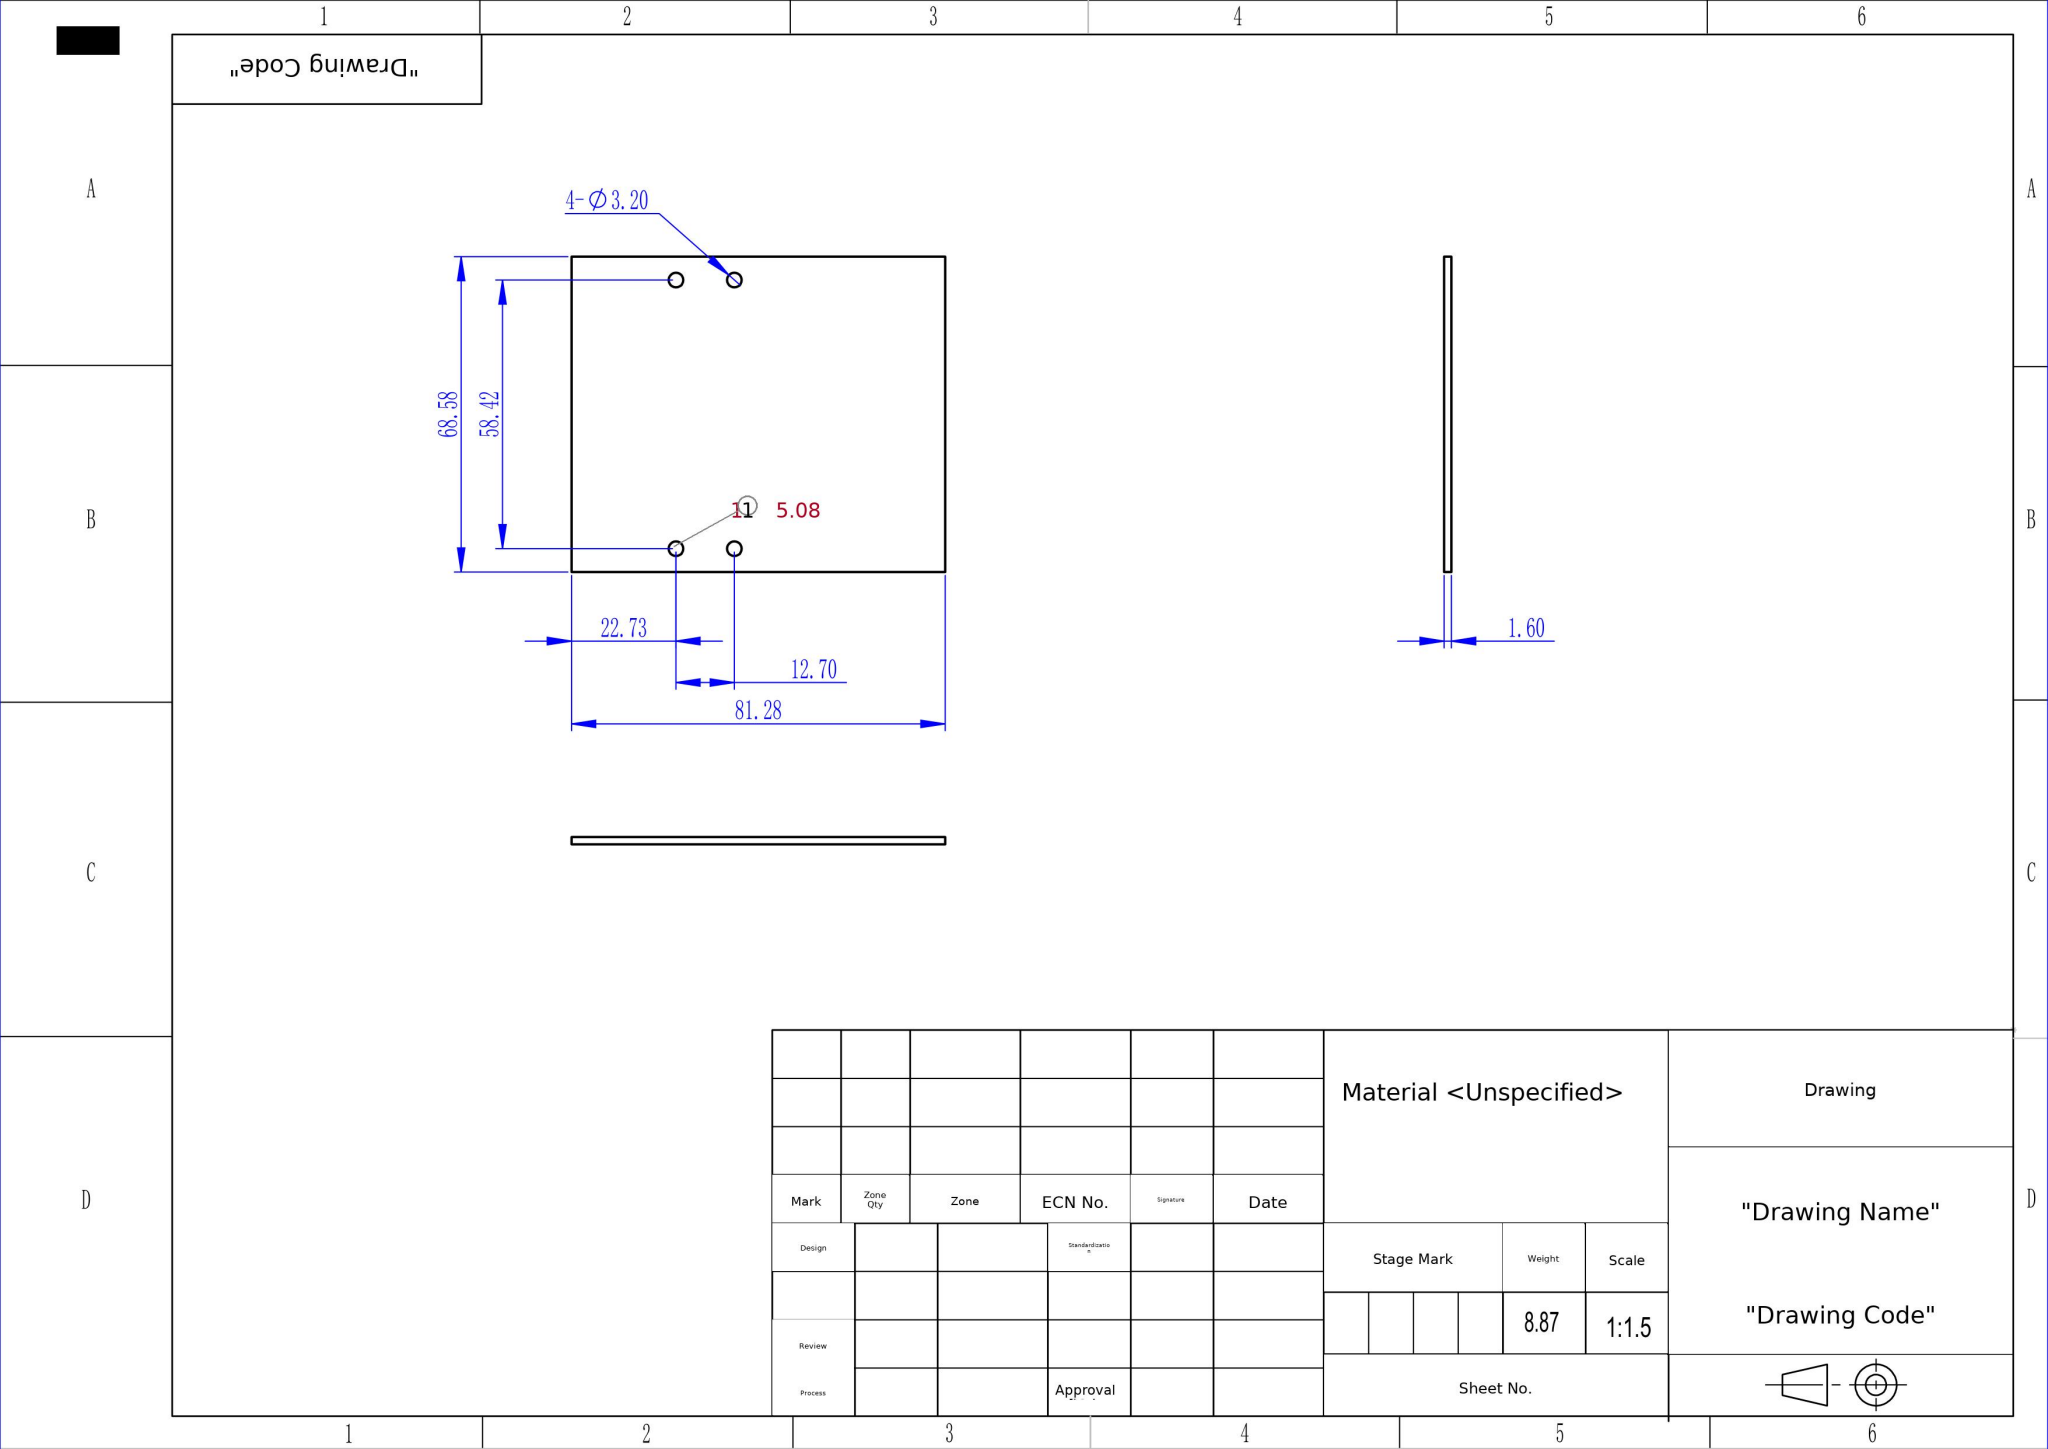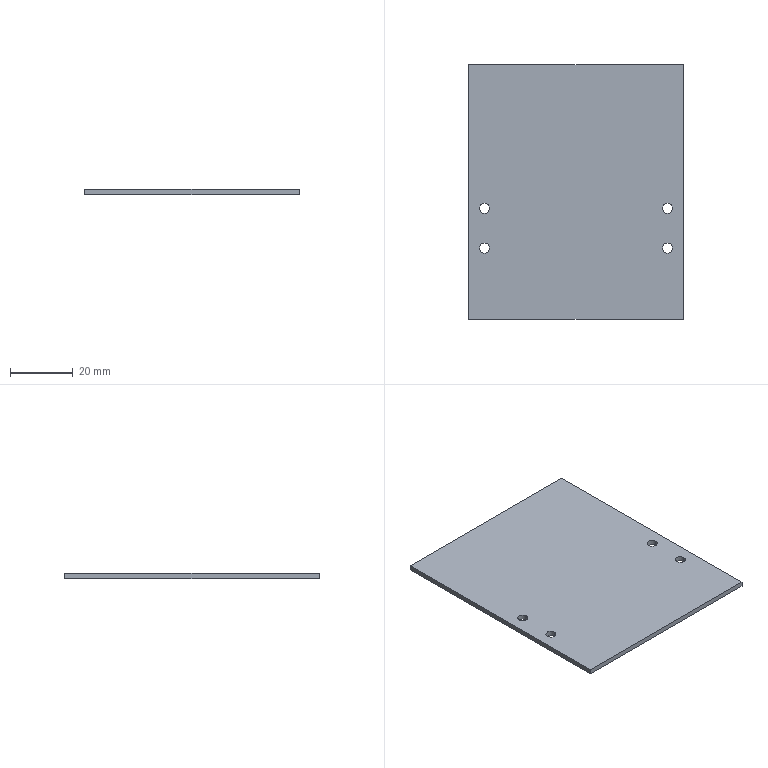Part | SolidWorks | mm | material Unspecified | 1 solid | 14 faces | box 68.58 x 81.28 x 1.6 mm | volume 8867 mm3 | cylinder 8 | plane 6 | commonest cylinder face diameters 3.2 x8
build123d program:
from build123d import *

# Parameters (mm, degrees)
SKETCH1_W           = 68.58
SKETCH1_H           = 81.28
SKETCH1_R           = 1.6
BOSS_EXTRUDE1_DEPTH = 1.6


with BuildPart() as part:
    # Sketch1 → Boss-Extrude1 (new body)
    with BuildSketch(Plane.XY):
        with Locations((0, 11.56)):
            Rectangle(SKETCH1_W, SKETCH1_H)
        with Locations((-29.21, 6.35)):
            Circle(SKETCH1_R, mode=Mode.SUBTRACT)
        with Locations((29.21, 6.35)):
            Circle(SKETCH1_R, mode=Mode.SUBTRACT)
        with Locations((29.21, -6.35)):
            Circle(SKETCH1_R, mode=Mode.SUBTRACT)
        with Locations((-29.21, -6.35)):
            Circle(SKETCH1_R, mode=Mode.SUBTRACT)
    extrude(amount=BOSS_EXTRUDE1_DEPTH)


solid = part.part
STEP:
#1=CARTESIAN_POINT('',(-30.81,-6.35,1.6));
#2=VERTEX_POINT('',#1);
#3=CARTESIAN_POINT('',(-27.61,-6.35,1.6));
#4=VERTEX_POINT('',#3);
#5=CARTESIAN_POINT('',(-29.21,-6.35,1.6));
#6=DIRECTION('',(0.,0.,1.));
#7=DIRECTION('',(1.,0.,0.));
#8=AXIS2_PLACEMENT_3D('',#5,#6,#7);
#9=CIRCLE('',#8,1.6);
#10=EDGE_CURVE('',#2,#4,#9,.T.);
#11=ORIENTED_EDGE('',*,*,#10,.T.);
#12=CARTESIAN_POINT('',(-27.61,-6.35,0.));
#13=VERTEX_POINT('',#12);
#14=CARTESIAN_POINT('',(-27.61,-6.35,1.6));
#15=DIRECTION('',(0.,0.,-1.));
#16=VECTOR('',#15,1000.);
#17=LINE('',#14,#16);
#18=EDGE_CURVE('',#4,#13,#17,.T.);
#19=ORIENTED_EDGE('',*,*,#18,.T.);
#20=CARTESIAN_POINT('',(-30.81,-6.35,0.));
#21=VERTEX_POINT('',#20);
#22=CARTESIAN_POINT('',(-29.21,-6.35,0.));
#23=DIRECTION('',(0.,0.,1.));
#24=DIRECTION('',(1.,0.,0.));
#25=AXIS2_PLACEMENT_3D('',#22,#23,#24);
#26=CIRCLE('',#25,1.6);
#27=EDGE_CURVE('',#21,#13,#26,.T.);
#28=ORIENTED_EDGE('',*,*,#27,.F.);
#29=CARTESIAN_POINT('',(-30.81,-6.35,1.6));
#30=DIRECTION('',(0.,0.,-1.));
#31=VECTOR('',#30,1000.);
#32=LINE('',#29,#31);
#33=EDGE_CURVE('',#2,#21,#32,.T.);
#34=ORIENTED_EDGE('',*,*,#33,.F.);
#35=EDGE_LOOP('',(#11,#19,#28,#34));
#36=FACE_OUTER_BOUND('',#35,.T.);
#37=CARTESIAN_POINT('',(-29.21,-6.35,1.6));
#38=DIRECTION('',(0.,0.,-1.));
#39=DIRECTION('',(-1.,0.,0.));
#40=AXIS2_PLACEMENT_3D('',#37,#38,#39);
#41=CYLINDRICAL_SURFACE('',#40,1.6);
#42=ADVANCED_FACE('',(#36),#41,.F.);
#43=CARTESIAN_POINT('',(27.61,-6.35,1.6));
#44=VERTEX_POINT('',#43);
#45=CARTESIAN_POINT('',(30.81,-6.35,1.6));
#46=VERTEX_POINT('',#45);
#47=CARTESIAN_POINT('',(29.21,-6.35,1.6));
#48=DIRECTION('',(0.,0.,1.));
#49=DIRECTION('',(1.,0.,0.));
#50=AXIS2_PLACEMENT_3D('',#47,#48,#49);
#51=CIRCLE('',#50,1.6);
#52=EDGE_CURVE('',#44,#46,#51,.T.);
#53=ORIENTED_EDGE('',*,*,#52,.T.);
#54=CARTESIAN_POINT('',(30.81,-6.35,0.));
#55=VERTEX_POINT('',#54);
#56=CARTESIAN_POINT('',(30.81,-6.35,1.6));
#57=DIRECTION('',(0.,0.,-1.));
#58=VECTOR('',#57,1000.);
#59=LINE('',#56,#58);
#60=EDGE_CURVE('',#46,#55,#59,.T.);
#61=ORIENTED_EDGE('',*,*,#60,.T.);
#62=CARTESIAN_POINT('',(27.61,-6.35,0.));
#63=VERTEX_POINT('',#62);
#64=CARTESIAN_POINT('',(29.21,-6.35,0.));
#65=DIRECTION('',(0.,0.,1.));
#66=DIRECTION('',(1.,0.,0.));
#67=AXIS2_PLACEMENT_3D('',#64,#65,#66);
#68=CIRCLE('',#67,1.6);
#69=EDGE_CURVE('',#63,#55,#68,.T.);
#70=ORIENTED_EDGE('',*,*,#69,.F.);
#71=CARTESIAN_POINT('',(27.61,-6.35,1.6));
#72=DIRECTION('',(0.,0.,-1.));
#73=VECTOR('',#72,1000.);
#74=LINE('',#71,#73);
#75=EDGE_CURVE('',#44,#63,#74,.T.);
#76=ORIENTED_EDGE('',*,*,#75,.F.);
#77=EDGE_LOOP('',(#53,#61,#70,#76));
#78=FACE_OUTER_BOUND('',#77,.T.);
#79=CARTESIAN_POINT('',(29.21,-6.35,1.6));
#80=DIRECTION('',(0.,0.,-1.));
#81=DIRECTION('',(-1.,0.,0.));
#82=AXIS2_PLACEMENT_3D('',#79,#80,#81);
#83=CYLINDRICAL_SURFACE('',#82,1.6);
#84=ADVANCED_FACE('',(#78),#83,.F.);
#85=CARTESIAN_POINT('',(27.61,6.35,1.6));
#86=VERTEX_POINT('',#85);
#87=CARTESIAN_POINT('',(30.81,6.35,1.6));
#88=VERTEX_POINT('',#87);
#89=CARTESIAN_POINT('',(29.21,6.35,1.6));
#90=DIRECTION('',(0.,0.,1.));
#91=DIRECTION('',(1.,0.,0.));
#92=AXIS2_PLACEMENT_3D('',#89,#90,#91);
#93=CIRCLE('',#92,1.6);
#94=EDGE_CURVE('',#86,#88,#93,.T.);
#95=ORIENTED_EDGE('',*,*,#94,.T.);
#96=CARTESIAN_POINT('',(30.81,6.35,0.));
#97=VERTEX_POINT('',#96);
#98=CARTESIAN_POINT('',(30.81,6.35,1.6));
#99=DIRECTION('',(0.,0.,-1.));
#100=VECTOR('',#99,1000.);
#101=LINE('',#98,#100);
#102=EDGE_CURVE('',#88,#97,#101,.T.);
#103=ORIENTED_EDGE('',*,*,#102,.T.);
#104=CARTESIAN_POINT('',(27.61,6.35,0.));
#105=VERTEX_POINT('',#104);
#106=CARTESIAN_POINT('',(29.21,6.35,0.));
#107=DIRECTION('',(0.,0.,1.));
#108=DIRECTION('',(1.,0.,0.));
#109=AXIS2_PLACEMENT_3D('',#106,#107,#108);
#110=CIRCLE('',#109,1.6);
#111=EDGE_CURVE('',#105,#97,#110,.T.);
#112=ORIENTED_EDGE('',*,*,#111,.F.);
#113=CARTESIAN_POINT('',(27.61,6.35,1.6));
#114=DIRECTION('',(0.,0.,-1.));
#115=VECTOR('',#114,1000.);
#116=LINE('',#113,#115);
#117=EDGE_CURVE('',#86,#105,#116,.T.);
#118=ORIENTED_EDGE('',*,*,#117,.F.);
#119=EDGE_LOOP('',(#95,#103,#112,#118));
#120=FACE_OUTER_BOUND('',#119,.T.);
#121=CARTESIAN_POINT('',(29.21,6.35,1.6));
#122=DIRECTION('',(0.,0.,-1.));
#123=DIRECTION('',(-1.,0.,0.));
#124=AXIS2_PLACEMENT_3D('',#121,#122,#123);
#125=CYLINDRICAL_SURFACE('',#124,1.6);
#126=ADVANCED_FACE('',(#120),#125,.F.);
#127=CARTESIAN_POINT('',(-30.81,6.35,1.6));
#128=VERTEX_POINT('',#127);
#129=CARTESIAN_POINT('',(-27.61,6.35,1.6));
#130=VERTEX_POINT('',#129);
#131=CARTESIAN_POINT('',(-29.21,6.35,1.6));
#132=DIRECTION('',(0.,0.,1.));
#133=DIRECTION('',(1.,0.,0.));
#134=AXIS2_PLACEMENT_3D('',#131,#132,#133);
#135=CIRCLE('',#134,1.6);
#136=EDGE_CURVE('',#128,#130,#135,.T.);
#137=ORIENTED_EDGE('',*,*,#136,.T.);
#138=CARTESIAN_POINT('',(-27.61,6.35,0.));
#139=VERTEX_POINT('',#138);
#140=CARTESIAN_POINT('',(-27.61,6.35,1.6));
#141=DIRECTION('',(0.,0.,-1.));
#142=VECTOR('',#141,1000.);
#143=LINE('',#140,#142);
#144=EDGE_CURVE('',#130,#139,#143,.T.);
#145=ORIENTED_EDGE('',*,*,#144,.T.);
#146=CARTESIAN_POINT('',(-30.81,6.35,0.));
#147=VERTEX_POINT('',#146);
#148=CARTESIAN_POINT('',(-29.21,6.35,0.));
#149=DIRECTION('',(0.,0.,1.));
#150=DIRECTION('',(1.,0.,0.));
#151=AXIS2_PLACEMENT_3D('',#148,#149,#150);
#152=CIRCLE('',#151,1.6);
#153=EDGE_CURVE('',#147,#139,#152,.T.);
#154=ORIENTED_EDGE('',*,*,#153,.F.);
#155=CARTESIAN_POINT('',(-30.81,6.35,1.6));
#156=DIRECTION('',(0.,0.,-1.));
#157=VECTOR('',#156,1000.);
#158=LINE('',#155,#157);
#159=EDGE_CURVE('',#128,#147,#158,.T.);
#160=ORIENTED_EDGE('',*,*,#159,.F.);
#161=EDGE_LOOP('',(#137,#145,#154,#160));
#162=FACE_OUTER_BOUND('',#161,.T.);
#163=CARTESIAN_POINT('',(-29.21,6.35,1.6));
#164=DIRECTION('',(0.,0.,-1.));
#165=DIRECTION('',(-1.,0.,0.));
#166=AXIS2_PLACEMENT_3D('',#163,#164,#165);
#167=CYLINDRICAL_SURFACE('',#166,1.6);
#168=ADVANCED_FACE('',(#162),#167,.F.);
#169=CARTESIAN_POINT('',(34.29,-29.08,1.6));
#170=VERTEX_POINT('',#169);
#171=CARTESIAN_POINT('',(34.29,52.2,1.6));
#172=VERTEX_POINT('',#171);
#173=CARTESIAN_POINT('',(34.29,-29.08,1.6));
#174=DIRECTION('',(0.,1.,0.));
#175=VECTOR('',#174,1000.);
#176=LINE('',#173,#175);
#177=EDGE_CURVE('',#170,#172,#176,.T.);
#178=ORIENTED_EDGE('',*,*,#177,.T.);
#179=CARTESIAN_POINT('',(-34.29,52.2,1.6));
#180=VERTEX_POINT('',#179);
#181=CARTESIAN_POINT('',(-34.29,52.2,1.6));
#182=DIRECTION('',(-1.,0.,0.));
#183=VECTOR('',#182,1000.);
#184=LINE('',#181,#183);
#185=EDGE_CURVE('',#172,#180,#184,.T.);
#186=ORIENTED_EDGE('',*,*,#185,.T.);
#187=CARTESIAN_POINT('',(-34.29,-29.08,1.6));
#188=VERTEX_POINT('',#187);
#189=CARTESIAN_POINT('',(-34.29,-29.08,1.6));
#190=DIRECTION('',(0.,-1.,0.));
#191=VECTOR('',#190,1000.);
#192=LINE('',#189,#191);
#193=EDGE_CURVE('',#180,#188,#192,.T.);
#194=ORIENTED_EDGE('',*,*,#193,.T.);
#195=CARTESIAN_POINT('',(-34.29,-29.08,1.6));
#196=DIRECTION('',(1.,0.,0.));
#197=VECTOR('',#196,1000.);
#198=LINE('',#195,#197);
#199=EDGE_CURVE('',#188,#170,#198,.T.);
#200=ORIENTED_EDGE('',*,*,#199,.T.);
#201=EDGE_LOOP('',(#178,#186,#194,#200));
#202=FACE_OUTER_BOUND('',#201,.T.);
#203=ORIENTED_EDGE('',*,*,#136,.F.);
#204=CARTESIAN_POINT('',(-29.21,6.35,1.6));
#205=DIRECTION('',(0.,0.,1.));
#206=DIRECTION('',(1.,0.,0.));
#207=AXIS2_PLACEMENT_3D('',#204,#205,#206);
#208=CIRCLE('',#207,1.6);
#209=EDGE_CURVE('',#130,#128,#208,.T.);
#210=ORIENTED_EDGE('',*,*,#209,.F.);
#211=EDGE_LOOP('',(#203,#210));
#212=FACE_BOUND('',#211,.T.);
#213=ORIENTED_EDGE('',*,*,#94,.F.);
#214=CARTESIAN_POINT('',(29.21,6.35,1.6));
#215=DIRECTION('',(0.,0.,1.));
#216=DIRECTION('',(1.,0.,0.));
#217=AXIS2_PLACEMENT_3D('',#214,#215,#216);
#218=CIRCLE('',#217,1.6);
#219=EDGE_CURVE('',#88,#86,#218,.T.);
#220=ORIENTED_EDGE('',*,*,#219,.F.);
#221=EDGE_LOOP('',(#213,#220));
#222=FACE_BOUND('',#221,.T.);
#223=ORIENTED_EDGE('',*,*,#52,.F.);
#224=CARTESIAN_POINT('',(29.21,-6.35,1.6));
#225=DIRECTION('',(0.,0.,1.));
#226=DIRECTION('',(1.,0.,0.));
#227=AXIS2_PLACEMENT_3D('',#224,#225,#226);
#228=CIRCLE('',#227,1.6);
#229=EDGE_CURVE('',#46,#44,#228,.T.);
#230=ORIENTED_EDGE('',*,*,#229,.F.);
#231=EDGE_LOOP('',(#223,#230));
#232=FACE_BOUND('',#231,.T.);
#233=ORIENTED_EDGE('',*,*,#10,.F.);
#234=CARTESIAN_POINT('',(-29.21,-6.35,1.6));
#235=DIRECTION('',(0.,0.,1.));
#236=DIRECTION('',(1.,0.,0.));
#237=AXIS2_PLACEMENT_3D('',#234,#235,#236);
#238=CIRCLE('',#237,1.6);
#239=EDGE_CURVE('',#4,#2,#238,.T.);
#240=ORIENTED_EDGE('',*,*,#239,.F.);
#241=EDGE_LOOP('',(#233,#240));
#242=FACE_BOUND('',#241,.T.);
#243=CARTESIAN_POINT('',(0.,0.,1.6));
#244=DIRECTION('',(0.,0.,-1.));
#245=DIRECTION('',(-1.,0.,0.));
#246=AXIS2_PLACEMENT_3D('',#243,#244,#245);
#247=PLANE('',#246);
#248=ADVANCED_FACE('',(#202,#212,#222,#232,#242),#247,.F.);
#249=ORIENTED_EDGE('',*,*,#69,.T.);
#250=CARTESIAN_POINT('',(29.21,-6.35,0.));
#251=DIRECTION('',(0.,0.,1.));
#252=DIRECTION('',(1.,0.,0.));
#253=AXIS2_PLACEMENT_3D('',#250,#251,#252);
#254=CIRCLE('',#253,1.6);
#255=EDGE_CURVE('',#55,#63,#254,.T.);
#256=ORIENTED_EDGE('',*,*,#255,.T.);
#257=EDGE_LOOP('',(#249,#256));
#258=FACE_BOUND('',#257,.T.);
#259=ORIENTED_EDGE('',*,*,#153,.T.);
#260=CARTESIAN_POINT('',(-29.21,6.35,0.));
#261=DIRECTION('',(0.,0.,1.));
#262=DIRECTION('',(1.,0.,0.));
#263=AXIS2_PLACEMENT_3D('',#260,#261,#262);
#264=CIRCLE('',#263,1.6);
#265=EDGE_CURVE('',#139,#147,#264,.T.);
#266=ORIENTED_EDGE('',*,*,#265,.T.);
#267=EDGE_LOOP('',(#259,#266));
#268=FACE_BOUND('',#267,.T.);
#269=CARTESIAN_POINT('',(34.29,-29.08,0.));
#270=VERTEX_POINT('',#269);
#271=CARTESIAN_POINT('',(34.29,52.2,0.));
#272=VERTEX_POINT('',#271);
#273=CARTESIAN_POINT('',(34.29,-29.08,0.));
#274=DIRECTION('',(0.,1.,0.));
#275=VECTOR('',#274,1000.);
#276=LINE('',#273,#275);
#277=EDGE_CURVE('',#270,#272,#276,.T.);
#278=ORIENTED_EDGE('',*,*,#277,.F.);
#279=CARTESIAN_POINT('',(-34.29,-29.08,0.));
#280=VERTEX_POINT('',#279);
#281=CARTESIAN_POINT('',(-34.29,-29.08,0.));
#282=DIRECTION('',(1.,0.,0.));
#283=VECTOR('',#282,1000.);
#284=LINE('',#281,#283);
#285=EDGE_CURVE('',#280,#270,#284,.T.);
#286=ORIENTED_EDGE('',*,*,#285,.F.);
#287=CARTESIAN_POINT('',(-34.29,52.2,0.));
#288=VERTEX_POINT('',#287);
#289=CARTESIAN_POINT('',(-34.29,-29.08,0.));
#290=DIRECTION('',(0.,-1.,0.));
#291=VECTOR('',#290,1000.);
#292=LINE('',#289,#291);
#293=EDGE_CURVE('',#288,#280,#292,.T.);
#294=ORIENTED_EDGE('',*,*,#293,.F.);
#295=CARTESIAN_POINT('',(-34.29,52.2,0.));
#296=DIRECTION('',(-1.,0.,0.));
#297=VECTOR('',#296,1000.);
#298=LINE('',#295,#297);
#299=EDGE_CURVE('',#272,#288,#298,.T.);
#300=ORIENTED_EDGE('',*,*,#299,.F.);
#301=EDGE_LOOP('',(#278,#286,#294,#300));
#302=FACE_OUTER_BOUND('',#301,.T.);
#303=ORIENTED_EDGE('',*,*,#111,.T.);
#304=CARTESIAN_POINT('',(29.21,6.35,0.));
#305=DIRECTION('',(0.,0.,1.));
#306=DIRECTION('',(1.,0.,0.));
#307=AXIS2_PLACEMENT_3D('',#304,#305,#306);
#308=CIRCLE('',#307,1.6);
#309=EDGE_CURVE('',#97,#105,#308,.T.);
#310=ORIENTED_EDGE('',*,*,#309,.T.);
#311=EDGE_LOOP('',(#303,#310));
#312=FACE_BOUND('',#311,.T.);
#313=ORIENTED_EDGE('',*,*,#27,.T.);
#314=CARTESIAN_POINT('',(-29.21,-6.35,0.));
#315=DIRECTION('',(0.,0.,1.));
#316=DIRECTION('',(1.,0.,0.));
#317=AXIS2_PLACEMENT_3D('',#314,#315,#316);
#318=CIRCLE('',#317,1.6);
#319=EDGE_CURVE('',#13,#21,#318,.T.);
#320=ORIENTED_EDGE('',*,*,#319,.T.);
#321=EDGE_LOOP('',(#313,#320));
#322=FACE_BOUND('',#321,.T.);
#323=CARTESIAN_POINT('',(0.,0.,0.));
#324=DIRECTION('',(0.,0.,-1.));
#325=DIRECTION('',(-1.,0.,0.));
#326=AXIS2_PLACEMENT_3D('',#323,#324,#325);
#327=PLANE('',#326);
#328=ADVANCED_FACE('',(#258,#268,#302,#312,#322),#327,.T.);
#329=ORIENTED_EDGE('',*,*,#277,.T.);
#330=CARTESIAN_POINT('',(34.29,52.2,1.6));
#331=DIRECTION('',(0.,0.,-1.));
#332=VECTOR('',#331,1000.);
#333=LINE('',#330,#332);
#334=EDGE_CURVE('',#172,#272,#333,.T.);
#335=ORIENTED_EDGE('',*,*,#334,.F.);
#336=ORIENTED_EDGE('',*,*,#177,.F.);
#337=CARTESIAN_POINT('',(34.29,-29.08,1.6));
#338=DIRECTION('',(0.,0.,-1.));
#339=VECTOR('',#338,1000.);
#340=LINE('',#337,#339);
#341=EDGE_CURVE('',#170,#270,#340,.T.);
#342=ORIENTED_EDGE('',*,*,#341,.T.);
#343=EDGE_LOOP('',(#329,#335,#336,#342));
#344=FACE_OUTER_BOUND('',#343,.T.);
#345=CARTESIAN_POINT('',(34.29,-29.08,1.6));
#346=DIRECTION('',(-1.,0.,0.));
#347=DIRECTION('',(0.,0.,1.));
#348=AXIS2_PLACEMENT_3D('',#345,#346,#347);
#349=PLANE('',#348);
#350=ADVANCED_FACE('',(#344),#349,.F.);
#351=ORIENTED_EDGE('',*,*,#299,.T.);
#352=CARTESIAN_POINT('',(-34.29,52.2,1.6));
#353=DIRECTION('',(0.,0.,-1.));
#354=VECTOR('',#353,1000.);
#355=LINE('',#352,#354);
#356=EDGE_CURVE('',#180,#288,#355,.T.);
#357=ORIENTED_EDGE('',*,*,#356,.F.);
#358=ORIENTED_EDGE('',*,*,#185,.F.);
#359=ORIENTED_EDGE('',*,*,#334,.T.);
#360=EDGE_LOOP('',(#351,#357,#358,#359));
#361=FACE_OUTER_BOUND('',#360,.T.);
#362=CARTESIAN_POINT('',(-34.29,52.2,1.6));
#363=DIRECTION('',(0.,-1.,0.));
#364=DIRECTION('',(0.,0.,-1.));
#365=AXIS2_PLACEMENT_3D('',#362,#363,#364);
#366=PLANE('',#365);
#367=ADVANCED_FACE('',(#361),#366,.F.);
#368=ORIENTED_EDGE('',*,*,#293,.T.);
#369=CARTESIAN_POINT('',(-34.29,-29.08,1.6));
#370=DIRECTION('',(0.,0.,-1.));
#371=VECTOR('',#370,1000.);
#372=LINE('',#369,#371);
#373=EDGE_CURVE('',#188,#280,#372,.T.);
#374=ORIENTED_EDGE('',*,*,#373,.F.);
#375=ORIENTED_EDGE('',*,*,#193,.F.);
#376=ORIENTED_EDGE('',*,*,#356,.T.);
#377=EDGE_LOOP('',(#368,#374,#375,#376));
#378=FACE_OUTER_BOUND('',#377,.T.);
#379=CARTESIAN_POINT('',(-34.29,-29.08,1.6));
#380=DIRECTION('',(1.,0.,0.));
#381=DIRECTION('',(0.,0.,-1.));
#382=AXIS2_PLACEMENT_3D('',#379,#380,#381);
#383=PLANE('',#382);
#384=ADVANCED_FACE('',(#378),#383,.F.);
#385=ORIENTED_EDGE('',*,*,#285,.T.);
#386=ORIENTED_EDGE('',*,*,#341,.F.);
#387=ORIENTED_EDGE('',*,*,#199,.F.);
#388=ORIENTED_EDGE('',*,*,#373,.T.);
#389=EDGE_LOOP('',(#385,#386,#387,#388));
#390=FACE_OUTER_BOUND('',#389,.T.);
#391=CARTESIAN_POINT('',(-34.29,-29.08,1.6));
#392=DIRECTION('',(0.,1.,0.));
#393=DIRECTION('',(0.,0.,1.));
#394=AXIS2_PLACEMENT_3D('',#391,#392,#393);
#395=PLANE('',#394);
#396=ADVANCED_FACE('',(#390),#395,.F.);
#397=ORIENTED_EDGE('',*,*,#144,.F.);
#398=ORIENTED_EDGE('',*,*,#209,.T.);
#399=ORIENTED_EDGE('',*,*,#159,.T.);
#400=ORIENTED_EDGE('',*,*,#265,.F.);
#401=EDGE_LOOP('',(#397,#398,#399,#400));
#402=FACE_OUTER_BOUND('',#401,.T.);
#403=CARTESIAN_POINT('',(-29.21,6.35,1.6));
#404=DIRECTION('',(0.,0.,-1.));
#405=DIRECTION('',(-1.,0.,0.));
#406=AXIS2_PLACEMENT_3D('',#403,#404,#405);
#407=CYLINDRICAL_SURFACE('',#406,1.6);
#408=ADVANCED_FACE('',(#402),#407,.F.);
#409=ORIENTED_EDGE('',*,*,#102,.F.);
#410=ORIENTED_EDGE('',*,*,#219,.T.);
#411=ORIENTED_EDGE('',*,*,#117,.T.);
#412=ORIENTED_EDGE('',*,*,#309,.F.);
#413=EDGE_LOOP('',(#409,#410,#411,#412));
#414=FACE_OUTER_BOUND('',#413,.T.);
#415=CARTESIAN_POINT('',(29.21,6.35,1.6));
#416=DIRECTION('',(0.,0.,-1.));
#417=DIRECTION('',(-1.,0.,0.));
#418=AXIS2_PLACEMENT_3D('',#415,#416,#417);
#419=CYLINDRICAL_SURFACE('',#418,1.6);
#420=ADVANCED_FACE('',(#414),#419,.F.);
#421=ORIENTED_EDGE('',*,*,#60,.F.);
#422=ORIENTED_EDGE('',*,*,#229,.T.);
#423=ORIENTED_EDGE('',*,*,#75,.T.);
#424=ORIENTED_EDGE('',*,*,#255,.F.);
#425=EDGE_LOOP('',(#421,#422,#423,#424));
#426=FACE_OUTER_BOUND('',#425,.T.);
#427=CARTESIAN_POINT('',(29.21,-6.35,1.6));
#428=DIRECTION('',(0.,0.,-1.));
#429=DIRECTION('',(-1.,0.,0.));
#430=AXIS2_PLACEMENT_3D('',#427,#428,#429);
#431=CYLINDRICAL_SURFACE('',#430,1.6);
#432=ADVANCED_FACE('',(#426),#431,.F.);
#433=ORIENTED_EDGE('',*,*,#18,.F.);
#434=ORIENTED_EDGE('',*,*,#239,.T.);
#435=ORIENTED_EDGE('',*,*,#33,.T.);
#436=ORIENTED_EDGE('',*,*,#319,.F.);
#437=EDGE_LOOP('',(#433,#434,#435,#436));
#438=FACE_OUTER_BOUND('',#437,.T.);
#439=CARTESIAN_POINT('',(-29.21,-6.35,1.6));
#440=DIRECTION('',(0.,0.,-1.));
#441=DIRECTION('',(-1.,0.,0.));
#442=AXIS2_PLACEMENT_3D('',#439,#440,#441);
#443=CYLINDRICAL_SURFACE('',#442,1.6);
#444=ADVANCED_FACE('',(#438),#443,.F.);
#445=CLOSED_SHELL('',(#42,#84,#126,#168,#248,#328,#350,#367,#384,#396,#408,#420,#432,#444));
#446=MANIFOLD_SOLID_BREP('',#445);
#447=CARTESIAN_POINT('',(0.,0.,0.));
#448=DIRECTION('',(0.,0.,1.));
#449=DIRECTION('',(1.,0.,0.));
#450=AXIS2_PLACEMENT_3D('',#447,#448,#449);
#451=(LENGTH_UNIT()NAMED_UNIT(*)SI_UNIT(.MILLI.,.METRE.));
#452=UNCERTAINTY_MEASURE_WITH_UNIT(LENGTH_MEASURE(0.00001),#451,'','');
#453=(NAMED_UNIT(*)PLANE_ANGLE_UNIT()SI_UNIT($,.RADIAN.));
#454=(NAMED_UNIT(*)SI_UNIT($,.STERADIAN.)SOLID_ANGLE_UNIT());
#455=(GEOMETRIC_REPRESENTATION_CONTEXT(3)GLOBAL_UNCERTAINTY_ASSIGNED_CONTEXT((#452))GLOBAL_UNIT_ASSIGNED_CONTEXT((#451,#453,#454))REPRESENTATION_CONTEXT('',''));
#456=ADVANCED_BREP_SHAPE_REPRESENTATION('',(#446,#450),#455);